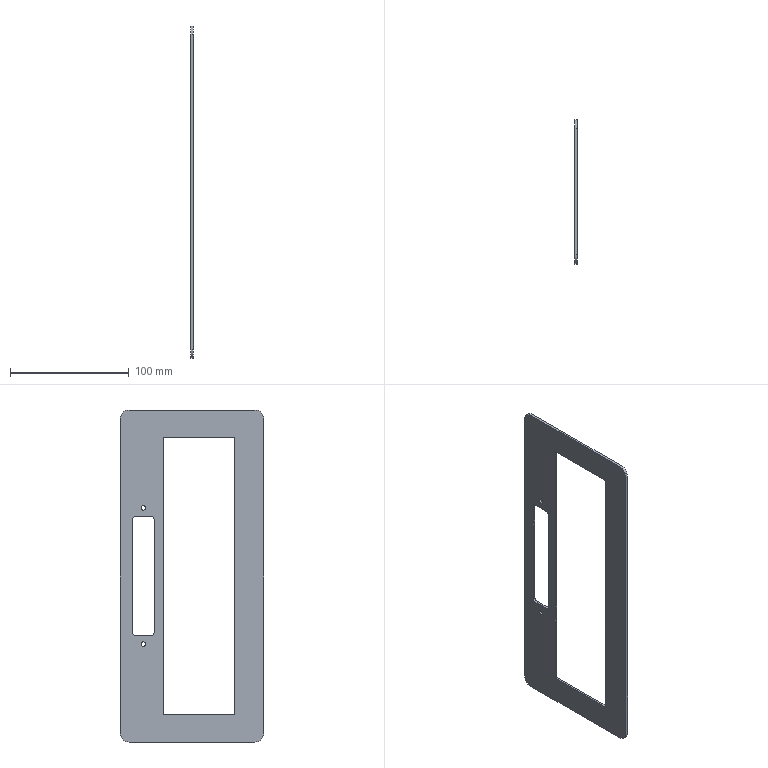Component | SolidWorks | YarnOutletAssembly-2_CashDispenserPanel-1 | 1 solid | 26 faces | box 2 x 121 x 280 mm | volume 35940 mm3 | plane 14 | cylinder 12 | commonest cylinder face diameters 4 x8 15 x4
STEP:
#1=CARTESIAN_POINT('',(-1.734,-15.239,2.343));
#2=VERTEX_POINT('',#1);
#3=CARTESIAN_POINT('',(-1.734,-15.239,2.185));
#4=VERTEX_POINT('',#3);
#5=CARTESIAN_POINT('',(-1.734,-15.239,2.264));
#6=DIRECTION('',(1.,0.,0.));
#7=DIRECTION('',(0.,0.,-1.));
#8=AXIS2_PLACEMENT_3D('',#5,#6,#7);
#9=CIRCLE('',#8,0.07874);
#10=EDGE_CURVE('',#2,#4,#9,.T.);
#11=ORIENTED_EDGE('',*,*,#10,.F.);
#12=CARTESIAN_POINT('',(-1.655,-15.239,2.343));
#13=VERTEX_POINT('',#12);
#14=CARTESIAN_POINT('',(-1.734,-15.239,2.343));
#15=DIRECTION('',(1.,0.,0.));
#16=VECTOR('',#15,39.37);
#17=LINE('',#14,#16);
#18=EDGE_CURVE('',#2,#13,#17,.T.);
#19=ORIENTED_EDGE('',*,*,#18,.T.);
#20=CARTESIAN_POINT('',(-1.655,-15.239,2.185));
#21=VERTEX_POINT('',#20);
#22=CARTESIAN_POINT('',(-1.655,-15.239,2.264));
#23=DIRECTION('',(1.,0.,0.));
#24=DIRECTION('',(0.,0.,-1.));
#25=AXIS2_PLACEMENT_3D('',#22,#23,#24);
#26=CIRCLE('',#25,0.07874);
#27=EDGE_CURVE('',#13,#21,#26,.T.);
#28=ORIENTED_EDGE('',*,*,#27,.T.);
#29=CARTESIAN_POINT('',(-1.734,-15.239,2.185));
#30=DIRECTION('',(1.,0.,0.));
#31=VECTOR('',#30,39.37);
#32=LINE('',#29,#31);
#33=EDGE_CURVE('',#4,#21,#32,.T.);
#34=ORIENTED_EDGE('',*,*,#33,.F.);
#35=EDGE_LOOP('',(#11,#19,#28,#34));
#36=FACE_OUTER_BOUND('',#35,.T.);
#37=CARTESIAN_POINT('',(-1.734,-15.239,2.264));
#38=DIRECTION('',(1.,0.,0.));
#39=DIRECTION('',(0.,0.,-1.));
#40=AXIS2_PLACEMENT_3D('',#37,#38,#39);
#41=CYLINDRICAL_SURFACE('',#40,0.07874);
#42=ADVANCED_FACE('',(#36),#41,.F.);
#43=CARTESIAN_POINT('',(-1.734,-15.239,-2.185));
#44=VERTEX_POINT('',#43);
#45=CARTESIAN_POINT('',(-1.734,-15.239,-2.343));
#46=VERTEX_POINT('',#45);
#47=CARTESIAN_POINT('',(-1.734,-15.239,-2.264));
#48=DIRECTION('',(1.,0.,0.));
#49=DIRECTION('',(0.,0.,-1.));
#50=AXIS2_PLACEMENT_3D('',#47,#48,#49);
#51=CIRCLE('',#50,0.07874);
#52=EDGE_CURVE('',#44,#46,#51,.T.);
#53=ORIENTED_EDGE('',*,*,#52,.F.);
#54=CARTESIAN_POINT('',(-1.655,-15.239,-2.185));
#55=VERTEX_POINT('',#54);
#56=CARTESIAN_POINT('',(-1.734,-15.239,-2.185));
#57=DIRECTION('',(1.,0.,0.));
#58=VECTOR('',#57,39.37);
#59=LINE('',#56,#58);
#60=EDGE_CURVE('',#44,#55,#59,.T.);
#61=ORIENTED_EDGE('',*,*,#60,.T.);
#62=CARTESIAN_POINT('',(-1.655,-15.239,-2.343));
#63=VERTEX_POINT('',#62);
#64=CARTESIAN_POINT('',(-1.655,-15.239,-2.264));
#65=DIRECTION('',(1.,0.,0.));
#66=DIRECTION('',(0.,0.,-1.));
#67=AXIS2_PLACEMENT_3D('',#64,#65,#66);
#68=CIRCLE('',#67,0.07874);
#69=EDGE_CURVE('',#55,#63,#68,.T.);
#70=ORIENTED_EDGE('',*,*,#69,.T.);
#71=CARTESIAN_POINT('',(-1.734,-15.239,-2.343));
#72=DIRECTION('',(1.,0.,0.));
#73=VECTOR('',#72,39.37);
#74=LINE('',#71,#73);
#75=EDGE_CURVE('',#46,#63,#74,.T.);
#76=ORIENTED_EDGE('',*,*,#75,.F.);
#77=EDGE_LOOP('',(#53,#61,#70,#76));
#78=FACE_OUTER_BOUND('',#77,.T.);
#79=CARTESIAN_POINT('',(-1.734,-15.239,-2.264));
#80=DIRECTION('',(1.,0.,0.));
#81=DIRECTION('',(0.,0.,-1.));
#82=AXIS2_PLACEMENT_3D('',#79,#80,#81);
#83=CYLINDRICAL_SURFACE('',#82,0.07874);
#84=ADVANCED_FACE('',(#78),#83,.F.);
#85=CARTESIAN_POINT('',(-1.655,-18.939,5.512));
#86=VERTEX_POINT('',#85);
#87=CARTESIAN_POINT('',(-1.655,-19.235,5.217));
#88=VERTEX_POINT('',#87);
#89=CARTESIAN_POINT('',(-1.655,-18.939,5.217));
#90=DIRECTION('',(1.,0.,0.));
#91=DIRECTION('',(0.,0.,-1.));
#92=AXIS2_PLACEMENT_3D('',#89,#90,#91);
#93=CIRCLE('',#92,0.2953);
#94=EDGE_CURVE('',#86,#88,#93,.T.);
#95=ORIENTED_EDGE('',*,*,#94,.F.);
#96=CARTESIAN_POINT('',(-1.734,-18.939,5.512));
#97=VERTEX_POINT('',#96);
#98=CARTESIAN_POINT('',(-1.734,-18.939,5.512));
#99=DIRECTION('',(1.,0.,0.));
#100=VECTOR('',#99,39.37);
#101=LINE('',#98,#100);
#102=EDGE_CURVE('',#97,#86,#101,.T.);
#103=ORIENTED_EDGE('',*,*,#102,.F.);
#104=CARTESIAN_POINT('',(-1.734,-19.235,5.217));
#105=VERTEX_POINT('',#104);
#106=CARTESIAN_POINT('',(-1.734,-18.939,5.217));
#107=DIRECTION('',(1.,0.,0.));
#108=DIRECTION('',(0.,0.,-1.));
#109=AXIS2_PLACEMENT_3D('',#106,#107,#108);
#110=CIRCLE('',#109,0.2953);
#111=EDGE_CURVE('',#97,#105,#110,.T.);
#112=ORIENTED_EDGE('',*,*,#111,.T.);
#113=CARTESIAN_POINT('',(-1.734,-19.235,5.217));
#114=DIRECTION('',(1.,0.,0.));
#115=VECTOR('',#114,39.37);
#116=LINE('',#113,#115);
#117=EDGE_CURVE('',#105,#88,#116,.T.);
#118=ORIENTED_EDGE('',*,*,#117,.T.);
#119=EDGE_LOOP('',(#95,#103,#112,#118));
#120=FACE_OUTER_BOUND('',#119,.T.);
#121=CARTESIAN_POINT('',(-1.734,-18.939,5.217));
#122=DIRECTION('',(1.,0.,0.));
#123=DIRECTION('',(0.,0.,-1.));
#124=AXIS2_PLACEMENT_3D('',#121,#122,#123);
#125=CYLINDRICAL_SURFACE('',#124,0.2953);
#126=ADVANCED_FACE('',(#120),#125,.T.);
#127=CARTESIAN_POINT('',(-1.655,-14.766,5.512));
#128=VERTEX_POINT('',#127);
#129=CARTESIAN_POINT('',(-1.655,-18.939,5.512));
#130=DIRECTION('',(0.,-1.,0.));
#131=VECTOR('',#130,39.37);
#132=LINE('',#129,#131);
#133=EDGE_CURVE('',#128,#86,#132,.T.);
#134=ORIENTED_EDGE('',*,*,#133,.F.);
#135=CARTESIAN_POINT('',(-1.734,-14.766,5.512));
#136=VERTEX_POINT('',#135);
#137=CARTESIAN_POINT('',(-1.734,-14.766,5.512));
#138=DIRECTION('',(1.,0.,0.));
#139=VECTOR('',#138,39.37);
#140=LINE('',#137,#139);
#141=EDGE_CURVE('',#136,#128,#140,.T.);
#142=ORIENTED_EDGE('',*,*,#141,.F.);
#143=CARTESIAN_POINT('',(-1.734,-18.939,5.512));
#144=DIRECTION('',(0.,-1.,0.));
#145=VECTOR('',#144,39.37);
#146=LINE('',#143,#145);
#147=EDGE_CURVE('',#136,#97,#146,.T.);
#148=ORIENTED_EDGE('',*,*,#147,.T.);
#149=ORIENTED_EDGE('',*,*,#102,.T.);
#150=EDGE_LOOP('',(#134,#142,#148,#149));
#151=FACE_OUTER_BOUND('',#150,.T.);
#152=CARTESIAN_POINT('',(-1.734,-18.939,5.512));
#153=DIRECTION('',(-0.,0.,1.));
#154=DIRECTION('',(1.,0.,0.));
#155=AXIS2_PLACEMENT_3D('',#152,#153,#154);
#156=PLANE('',#155);
#157=ADVANCED_FACE('',(#151),#156,.T.);
#158=CARTESIAN_POINT('',(-1.655,-14.471,5.217));
#159=VERTEX_POINT('',#158);
#160=CARTESIAN_POINT('',(-1.655,-14.766,5.217));
#161=DIRECTION('',(1.,0.,0.));
#162=DIRECTION('',(0.,0.,-1.));
#163=AXIS2_PLACEMENT_3D('',#160,#161,#162);
#164=CIRCLE('',#163,0.2953);
#165=EDGE_CURVE('',#159,#128,#164,.T.);
#166=ORIENTED_EDGE('',*,*,#165,.F.);
#167=CARTESIAN_POINT('',(-1.734,-14.471,5.217));
#168=VERTEX_POINT('',#167);
#169=CARTESIAN_POINT('',(-1.734,-14.471,5.217));
#170=DIRECTION('',(1.,0.,0.));
#171=VECTOR('',#170,39.37);
#172=LINE('',#169,#171);
#173=EDGE_CURVE('',#168,#159,#172,.T.);
#174=ORIENTED_EDGE('',*,*,#173,.F.);
#175=CARTESIAN_POINT('',(-1.734,-14.766,5.217));
#176=DIRECTION('',(1.,0.,0.));
#177=DIRECTION('',(0.,0.,-1.));
#178=AXIS2_PLACEMENT_3D('',#175,#176,#177);
#179=CIRCLE('',#178,0.2953);
#180=EDGE_CURVE('',#168,#136,#179,.T.);
#181=ORIENTED_EDGE('',*,*,#180,.T.);
#182=ORIENTED_EDGE('',*,*,#141,.T.);
#183=EDGE_LOOP('',(#166,#174,#181,#182));
#184=FACE_OUTER_BOUND('',#183,.T.);
#185=CARTESIAN_POINT('',(-1.734,-14.766,5.217));
#186=DIRECTION('',(1.,0.,0.));
#187=DIRECTION('',(0.,0.,-1.));
#188=AXIS2_PLACEMENT_3D('',#185,#186,#187);
#189=CYLINDRICAL_SURFACE('',#188,0.2953);
#190=ADVANCED_FACE('',(#184),#189,.T.);
#191=CARTESIAN_POINT('',(-1.655,-14.471,-5.217));
#192=VERTEX_POINT('',#191);
#193=CARTESIAN_POINT('',(-1.655,-14.471,5.217));
#194=DIRECTION('',(-0.,0.,1.));
#195=VECTOR('',#194,39.37);
#196=LINE('',#193,#195);
#197=EDGE_CURVE('',#192,#159,#196,.T.);
#198=ORIENTED_EDGE('',*,*,#197,.F.);
#199=CARTESIAN_POINT('',(-1.734,-14.471,-5.217));
#200=VERTEX_POINT('',#199);
#201=CARTESIAN_POINT('',(-1.734,-14.471,-5.217));
#202=DIRECTION('',(1.,0.,0.));
#203=VECTOR('',#202,39.37);
#204=LINE('',#201,#203);
#205=EDGE_CURVE('',#200,#192,#204,.T.);
#206=ORIENTED_EDGE('',*,*,#205,.F.);
#207=CARTESIAN_POINT('',(-1.734,-14.471,5.217));
#208=DIRECTION('',(-0.,0.,1.));
#209=VECTOR('',#208,39.37);
#210=LINE('',#207,#209);
#211=EDGE_CURVE('',#200,#168,#210,.T.);
#212=ORIENTED_EDGE('',*,*,#211,.T.);
#213=ORIENTED_EDGE('',*,*,#173,.T.);
#214=EDGE_LOOP('',(#198,#206,#212,#213));
#215=FACE_OUTER_BOUND('',#214,.T.);
#216=CARTESIAN_POINT('',(-1.734,-14.471,5.217));
#217=DIRECTION('',(-0.,1.,-0.));
#218=DIRECTION('',(1.,0.,0.));
#219=AXIS2_PLACEMENT_3D('',#216,#217,#218);
#220=PLANE('',#219);
#221=ADVANCED_FACE('',(#215),#220,.T.);
#222=CARTESIAN_POINT('',(-1.655,-14.766,-5.512));
#223=VERTEX_POINT('',#222);
#224=CARTESIAN_POINT('',(-1.655,-14.766,-5.217));
#225=DIRECTION('',(1.,0.,0.));
#226=DIRECTION('',(0.,0.,-1.));
#227=AXIS2_PLACEMENT_3D('',#224,#225,#226);
#228=CIRCLE('',#227,0.2953);
#229=EDGE_CURVE('',#223,#192,#228,.T.);
#230=ORIENTED_EDGE('',*,*,#229,.F.);
#231=CARTESIAN_POINT('',(-1.734,-14.766,-5.512));
#232=VERTEX_POINT('',#231);
#233=CARTESIAN_POINT('',(-1.734,-14.766,-5.512));
#234=DIRECTION('',(1.,0.,0.));
#235=VECTOR('',#234,39.37);
#236=LINE('',#233,#235);
#237=EDGE_CURVE('',#232,#223,#236,.T.);
#238=ORIENTED_EDGE('',*,*,#237,.F.);
#239=CARTESIAN_POINT('',(-1.734,-14.766,-5.217));
#240=DIRECTION('',(1.,0.,0.));
#241=DIRECTION('',(0.,0.,-1.));
#242=AXIS2_PLACEMENT_3D('',#239,#240,#241);
#243=CIRCLE('',#242,0.2953);
#244=EDGE_CURVE('',#232,#200,#243,.T.);
#245=ORIENTED_EDGE('',*,*,#244,.T.);
#246=ORIENTED_EDGE('',*,*,#205,.T.);
#247=EDGE_LOOP('',(#230,#238,#245,#246));
#248=FACE_OUTER_BOUND('',#247,.T.);
#249=CARTESIAN_POINT('',(-1.734,-14.766,-5.217));
#250=DIRECTION('',(1.,0.,0.));
#251=DIRECTION('',(0.,0.,-1.));
#252=AXIS2_PLACEMENT_3D('',#249,#250,#251);
#253=CYLINDRICAL_SURFACE('',#252,0.2953);
#254=ADVANCED_FACE('',(#248),#253,.T.);
#255=CARTESIAN_POINT('',(-1.655,-18.939,-5.512));
#256=VERTEX_POINT('',#255);
#257=CARTESIAN_POINT('',(-1.655,-18.939,-5.512));
#258=DIRECTION('',(-0.,1.,-0.));
#259=VECTOR('',#258,39.37);
#260=LINE('',#257,#259);
#261=EDGE_CURVE('',#256,#223,#260,.T.);
#262=ORIENTED_EDGE('',*,*,#261,.F.);
#263=CARTESIAN_POINT('',(-1.734,-18.939,-5.512));
#264=VERTEX_POINT('',#263);
#265=CARTESIAN_POINT('',(-1.734,-18.939,-5.512));
#266=DIRECTION('',(1.,0.,0.));
#267=VECTOR('',#266,39.37);
#268=LINE('',#265,#267);
#269=EDGE_CURVE('',#264,#256,#268,.T.);
#270=ORIENTED_EDGE('',*,*,#269,.F.);
#271=CARTESIAN_POINT('',(-1.734,-18.939,-5.512));
#272=DIRECTION('',(-0.,1.,-0.));
#273=VECTOR('',#272,39.37);
#274=LINE('',#271,#273);
#275=EDGE_CURVE('',#264,#232,#274,.T.);
#276=ORIENTED_EDGE('',*,*,#275,.T.);
#277=ORIENTED_EDGE('',*,*,#237,.T.);
#278=EDGE_LOOP('',(#262,#270,#276,#277));
#279=FACE_OUTER_BOUND('',#278,.T.);
#280=CARTESIAN_POINT('',(-1.734,-18.939,-5.512));
#281=DIRECTION('',(0.,-0.,-1.));
#282=DIRECTION('',(-1.,-0.,0.));
#283=AXIS2_PLACEMENT_3D('',#280,#281,#282);
#284=PLANE('',#283);
#285=ADVANCED_FACE('',(#279),#284,.T.);
#286=CARTESIAN_POINT('',(-1.655,-19.235,-5.217));
#287=VERTEX_POINT('',#286);
#288=CARTESIAN_POINT('',(-1.655,-18.939,-5.217));
#289=DIRECTION('',(1.,0.,0.));
#290=DIRECTION('',(0.,0.,-1.));
#291=AXIS2_PLACEMENT_3D('',#288,#289,#290);
#292=CIRCLE('',#291,0.2953);
#293=EDGE_CURVE('',#287,#256,#292,.T.);
#294=ORIENTED_EDGE('',*,*,#293,.F.);
#295=CARTESIAN_POINT('',(-1.734,-19.235,-5.217));
#296=VERTEX_POINT('',#295);
#297=CARTESIAN_POINT('',(-1.734,-19.235,-5.217));
#298=DIRECTION('',(1.,0.,0.));
#299=VECTOR('',#298,39.37);
#300=LINE('',#297,#299);
#301=EDGE_CURVE('',#296,#287,#300,.T.);
#302=ORIENTED_EDGE('',*,*,#301,.F.);
#303=CARTESIAN_POINT('',(-1.734,-18.939,-5.217));
#304=DIRECTION('',(1.,0.,0.));
#305=DIRECTION('',(0.,0.,-1.));
#306=AXIS2_PLACEMENT_3D('',#303,#304,#305);
#307=CIRCLE('',#306,0.2953);
#308=EDGE_CURVE('',#296,#264,#307,.T.);
#309=ORIENTED_EDGE('',*,*,#308,.T.);
#310=ORIENTED_EDGE('',*,*,#269,.T.);
#311=EDGE_LOOP('',(#294,#302,#309,#310));
#312=FACE_OUTER_BOUND('',#311,.T.);
#313=CARTESIAN_POINT('',(-1.734,-18.939,-5.217));
#314=DIRECTION('',(1.,0.,0.));
#315=DIRECTION('',(0.,0.,-1.));
#316=AXIS2_PLACEMENT_3D('',#313,#314,#315);
#317=CYLINDRICAL_SURFACE('',#316,0.2953);
#318=ADVANCED_FACE('',(#312),#317,.T.);
#319=CARTESIAN_POINT('',(-1.655,-19.235,5.217));
#320=DIRECTION('',(0.,-0.,-1.));
#321=VECTOR('',#320,39.37);
#322=LINE('',#319,#321);
#323=EDGE_CURVE('',#88,#287,#322,.T.);
#324=ORIENTED_EDGE('',*,*,#323,.F.);
#325=ORIENTED_EDGE('',*,*,#117,.F.);
#326=CARTESIAN_POINT('',(-1.734,-19.235,5.217));
#327=DIRECTION('',(0.,-0.,-1.));
#328=VECTOR('',#327,39.37);
#329=LINE('',#326,#328);
#330=EDGE_CURVE('',#105,#296,#329,.T.);
#331=ORIENTED_EDGE('',*,*,#330,.T.);
#332=ORIENTED_EDGE('',*,*,#301,.T.);
#333=EDGE_LOOP('',(#324,#325,#331,#332));
#334=FACE_OUTER_BOUND('',#333,.T.);
#335=CARTESIAN_POINT('',(-1.734,-19.235,5.217));
#336=DIRECTION('',(0.,-1.,0.));
#337=DIRECTION('',(-1.,-0.,0.));
#338=AXIS2_PLACEMENT_3D('',#335,#336,#337);
#339=PLANE('',#338);
#340=ADVANCED_FACE('',(#334),#339,.T.);
#341=CARTESIAN_POINT('',(-1.734,-15.239,2.264));
#342=DIRECTION('',(1.,0.,0.));
#343=DIRECTION('',(0.,0.,-1.));
#344=AXIS2_PLACEMENT_3D('',#341,#342,#343);
#345=CIRCLE('',#344,0.07874);
#346=EDGE_CURVE('',#4,#2,#345,.T.);
#347=ORIENTED_EDGE('',*,*,#346,.T.);
#348=ORIENTED_EDGE('',*,*,#10,.T.);
#349=EDGE_LOOP('',(#347,#348));
#350=FACE_BOUND('',#349,.T.);
#351=CARTESIAN_POINT('',(-1.734,-15.239,-2.264));
#352=DIRECTION('',(1.,0.,0.));
#353=DIRECTION('',(0.,0.,-1.));
#354=AXIS2_PLACEMENT_3D('',#351,#352,#353);
#355=CIRCLE('',#354,0.07874);
#356=EDGE_CURVE('',#46,#44,#355,.T.);
#357=ORIENTED_EDGE('',*,*,#356,.T.);
#358=ORIENTED_EDGE('',*,*,#52,.T.);
#359=EDGE_LOOP('',(#357,#358));
#360=FACE_BOUND('',#359,.T.);
#361=CARTESIAN_POINT('',(-1.734,-14.884,-1.89));
#362=VERTEX_POINT('',#361);
#363=CARTESIAN_POINT('',(-1.734,-14.884,1.89));
#364=VERTEX_POINT('',#363);
#365=CARTESIAN_POINT('',(-1.734,-14.884,-1.89));
#366=DIRECTION('',(-0.,0.,1.));
#367=VECTOR('',#366,39.37);
#368=LINE('',#365,#367);
#369=EDGE_CURVE('',#362,#364,#368,.T.);
#370=ORIENTED_EDGE('',*,*,#369,.T.);
#371=CARTESIAN_POINT('',(-1.734,-14.963,1.969));
#372=VERTEX_POINT('',#371);
#373=CARTESIAN_POINT('',(-1.734,-14.963,1.89));
#374=DIRECTION('',(1.,0.,0.));
#375=DIRECTION('',(0.,0.,-1.));
#376=AXIS2_PLACEMENT_3D('',#373,#374,#375);
#377=CIRCLE('',#376,0.07874);
#378=EDGE_CURVE('',#364,#372,#377,.T.);
#379=ORIENTED_EDGE('',*,*,#378,.T.);
#380=CARTESIAN_POINT('',(-1.734,-15.514,1.969));
#381=VERTEX_POINT('',#380);
#382=CARTESIAN_POINT('',(-1.734,-14.963,1.969));
#383=DIRECTION('',(0.,-1.,0.));
#384=VECTOR('',#383,39.37);
#385=LINE('',#382,#384);
#386=EDGE_CURVE('',#372,#381,#385,.T.);
#387=ORIENTED_EDGE('',*,*,#386,.T.);
#388=CARTESIAN_POINT('',(-1.734,-15.593,1.89));
#389=VERTEX_POINT('',#388);
#390=CARTESIAN_POINT('',(-1.734,-15.514,1.89));
#391=DIRECTION('',(1.,0.,0.));
#392=DIRECTION('',(0.,0.,-1.));
#393=AXIS2_PLACEMENT_3D('',#390,#391,#392);
#394=CIRCLE('',#393,0.07874);
#395=EDGE_CURVE('',#381,#389,#394,.T.);
#396=ORIENTED_EDGE('',*,*,#395,.T.);
#397=CARTESIAN_POINT('',(-1.734,-15.593,-1.89));
#398=VERTEX_POINT('',#397);
#399=CARTESIAN_POINT('',(-1.734,-15.593,1.89));
#400=DIRECTION('',(0.,-0.,-1.));
#401=VECTOR('',#400,39.37);
#402=LINE('',#399,#401);
#403=EDGE_CURVE('',#389,#398,#402,.T.);
#404=ORIENTED_EDGE('',*,*,#403,.T.);
#405=CARTESIAN_POINT('',(-1.734,-15.514,-1.969));
#406=VERTEX_POINT('',#405);
#407=CARTESIAN_POINT('',(-1.734,-15.514,-1.89));
#408=DIRECTION('',(1.,0.,0.));
#409=DIRECTION('',(0.,0.,-1.));
#410=AXIS2_PLACEMENT_3D('',#407,#408,#409);
#411=CIRCLE('',#410,0.07874);
#412=EDGE_CURVE('',#398,#406,#411,.T.);
#413=ORIENTED_EDGE('',*,*,#412,.T.);
#414=CARTESIAN_POINT('',(-1.734,-14.963,-1.969));
#415=VERTEX_POINT('',#414);
#416=CARTESIAN_POINT('',(-1.734,-15.514,-1.969));
#417=DIRECTION('',(-0.,1.,-0.));
#418=VECTOR('',#417,39.37);
#419=LINE('',#416,#418);
#420=EDGE_CURVE('',#406,#415,#419,.T.);
#421=ORIENTED_EDGE('',*,*,#420,.T.);
#422=CARTESIAN_POINT('',(-1.734,-14.963,-1.89));
#423=DIRECTION('',(1.,0.,0.));
#424=DIRECTION('',(0.,0.,-1.));
#425=AXIS2_PLACEMENT_3D('',#422,#423,#424);
#426=CIRCLE('',#425,0.07874);
#427=EDGE_CURVE('',#415,#362,#426,.T.);
#428=ORIENTED_EDGE('',*,*,#427,.T.);
#429=EDGE_LOOP('',(#370,#379,#387,#396,#404,#413,#421,#428));
#430=FACE_BOUND('',#429,.T.);
#431=CARTESIAN_POINT('',(-1.734,-18.27,-4.606));
#432=VERTEX_POINT('',#431);
#433=CARTESIAN_POINT('',(-1.734,-15.908,-4.606));
#434=VERTEX_POINT('',#433);
#435=CARTESIAN_POINT('',(-1.734,-18.27,-4.606));
#436=DIRECTION('',(-0.,1.,-0.));
#437=VECTOR('',#436,39.37);
#438=LINE('',#435,#437);
#439=EDGE_CURVE('',#432,#434,#438,.T.);
#440=ORIENTED_EDGE('',*,*,#439,.T.);
#441=CARTESIAN_POINT('',(-1.734,-15.908,4.606));
#442=VERTEX_POINT('',#441);
#443=CARTESIAN_POINT('',(-1.734,-15.908,-4.606));
#444=DIRECTION('',(-0.,0.,1.));
#445=VECTOR('',#444,39.37);
#446=LINE('',#443,#445);
#447=EDGE_CURVE('',#434,#442,#446,.T.);
#448=ORIENTED_EDGE('',*,*,#447,.T.);
#449=CARTESIAN_POINT('',(-1.734,-18.27,4.606));
#450=VERTEX_POINT('',#449);
#451=CARTESIAN_POINT('',(-1.734,-15.908,4.606));
#452=DIRECTION('',(0.,-1.,0.));
#453=VECTOR('',#452,39.37);
#454=LINE('',#451,#453);
#455=EDGE_CURVE('',#442,#450,#454,.T.);
#456=ORIENTED_EDGE('',*,*,#455,.T.);
#457=CARTESIAN_POINT('',(-1.734,-18.27,4.606));
#458=DIRECTION('',(0.,-0.,-1.));
#459=VECTOR('',#458,39.37);
#460=LINE('',#457,#459);
#461=EDGE_CURVE('',#450,#432,#460,.T.);
#462=ORIENTED_EDGE('',*,*,#461,.T.);
#463=EDGE_LOOP('',(#440,#448,#456,#462));
#464=FACE_BOUND('',#463,.T.);
#465=ORIENTED_EDGE('',*,*,#111,.F.);
#466=ORIENTED_EDGE('',*,*,#147,.F.);
#467=ORIENTED_EDGE('',*,*,#180,.F.);
#468=ORIENTED_EDGE('',*,*,#211,.F.);
#469=ORIENTED_EDGE('',*,*,#244,.F.);
#470=ORIENTED_EDGE('',*,*,#275,.F.);
#471=ORIENTED_EDGE('',*,*,#308,.F.);
#472=ORIENTED_EDGE('',*,*,#330,.F.);
#473=EDGE_LOOP('',(#465,#466,#467,#468,#469,#470,#471,#472));
#474=FACE_OUTER_BOUND('',#473,.T.);
#475=CARTESIAN_POINT('',(-1.734,-18.939,5.217));
#476=DIRECTION('',(1.,0.,0.));
#477=DIRECTION('',(0.,-0.,-1.));
#478=AXIS2_PLACEMENT_3D('',#475,#476,#477);
#479=PLANE('',#478);
#480=ADVANCED_FACE('',(#350,#360,#430,#464,#474),#479,.F.);
#481=CARTESIAN_POINT('',(-1.655,-15.239,2.264));
#482=DIRECTION('',(1.,0.,0.));
#483=DIRECTION('',(0.,0.,-1.));
#484=AXIS2_PLACEMENT_3D('',#481,#482,#483);
#485=CIRCLE('',#484,0.07874);
#486=EDGE_CURVE('',#21,#13,#485,.T.);
#487=ORIENTED_EDGE('',*,*,#486,.F.);
#488=ORIENTED_EDGE('',*,*,#27,.F.);
#489=EDGE_LOOP('',(#487,#488));
#490=FACE_BOUND('',#489,.T.);
#491=CARTESIAN_POINT('',(-1.655,-15.239,-2.264));
#492=DIRECTION('',(1.,0.,0.));
#493=DIRECTION('',(0.,0.,-1.));
#494=AXIS2_PLACEMENT_3D('',#491,#492,#493);
#495=CIRCLE('',#494,0.07874);
#496=EDGE_CURVE('',#63,#55,#495,.T.);
#497=ORIENTED_EDGE('',*,*,#496,.F.);
#498=ORIENTED_EDGE('',*,*,#69,.F.);
#499=EDGE_LOOP('',(#497,#498));
#500=FACE_BOUND('',#499,.T.);
#501=CARTESIAN_POINT('',(-1.655,-14.884,1.89));
#502=VERTEX_POINT('',#501);
#503=CARTESIAN_POINT('',(-1.655,-14.963,1.969));
#504=VERTEX_POINT('',#503);
#505=CARTESIAN_POINT('',(-1.655,-14.963,1.89));
#506=DIRECTION('',(1.,0.,0.));
#507=DIRECTION('',(0.,0.,-1.));
#508=AXIS2_PLACEMENT_3D('',#505,#506,#507);
#509=CIRCLE('',#508,0.07874);
#510=EDGE_CURVE('',#502,#504,#509,.T.);
#511=ORIENTED_EDGE('',*,*,#510,.F.);
#512=CARTESIAN_POINT('',(-1.655,-14.884,-1.89));
#513=VERTEX_POINT('',#512);
#514=CARTESIAN_POINT('',(-1.655,-14.884,-1.89));
#515=DIRECTION('',(-0.,0.,1.));
#516=VECTOR('',#515,39.37);
#517=LINE('',#514,#516);
#518=EDGE_CURVE('',#513,#502,#517,.T.);
#519=ORIENTED_EDGE('',*,*,#518,.F.);
#520=CARTESIAN_POINT('',(-1.655,-14.963,-1.969));
#521=VERTEX_POINT('',#520);
#522=CARTESIAN_POINT('',(-1.655,-14.963,-1.89));
#523=DIRECTION('',(1.,0.,0.));
#524=DIRECTION('',(0.,0.,-1.));
#525=AXIS2_PLACEMENT_3D('',#522,#523,#524);
#526=CIRCLE('',#525,0.07874);
#527=EDGE_CURVE('',#521,#513,#526,.T.);
#528=ORIENTED_EDGE('',*,*,#527,.F.);
#529=CARTESIAN_POINT('',(-1.655,-15.514,-1.969));
#530=VERTEX_POINT('',#529);
#531=CARTESIAN_POINT('',(-1.655,-15.514,-1.969));
#532=DIRECTION('',(-0.,1.,-0.));
#533=VECTOR('',#532,39.37);
#534=LINE('',#531,#533);
#535=EDGE_CURVE('',#530,#521,#534,.T.);
#536=ORIENTED_EDGE('',*,*,#535,.F.);
#537=CARTESIAN_POINT('',(-1.655,-15.593,-1.89));
#538=VERTEX_POINT('',#537);
#539=CARTESIAN_POINT('',(-1.655,-15.514,-1.89));
#540=DIRECTION('',(1.,0.,0.));
#541=DIRECTION('',(0.,0.,-1.));
#542=AXIS2_PLACEMENT_3D('',#539,#540,#541);
#543=CIRCLE('',#542,0.07874);
#544=EDGE_CURVE('',#538,#530,#543,.T.);
#545=ORIENTED_EDGE('',*,*,#544,.F.);
#546=CARTESIAN_POINT('',(-1.655,-15.593,1.89));
#547=VERTEX_POINT('',#546);
#548=CARTESIAN_POINT('',(-1.655,-15.593,1.89));
#549=DIRECTION('',(0.,-0.,-1.));
#550=VECTOR('',#549,39.37);
#551=LINE('',#548,#550);
#552=EDGE_CURVE('',#547,#538,#551,.T.);
#553=ORIENTED_EDGE('',*,*,#552,.F.);
#554=CARTESIAN_POINT('',(-1.655,-15.514,1.969));
#555=VERTEX_POINT('',#554);
#556=CARTESIAN_POINT('',(-1.655,-15.514,1.89));
#557=DIRECTION('',(1.,0.,0.));
#558=DIRECTION('',(0.,0.,-1.));
#559=AXIS2_PLACEMENT_3D('',#556,#557,#558);
#560=CIRCLE('',#559,0.07874);
#561=EDGE_CURVE('',#555,#547,#560,.T.);
#562=ORIENTED_EDGE('',*,*,#561,.F.);
#563=CARTESIAN_POINT('',(-1.655,-14.963,1.969));
#564=DIRECTION('',(0.,-1.,0.));
#565=VECTOR('',#564,39.37);
#566=LINE('',#563,#565);
#567=EDGE_CURVE('',#504,#555,#566,.T.);
#568=ORIENTED_EDGE('',*,*,#567,.F.);
#569=EDGE_LOOP('',(#511,#519,#528,#536,#545,#553,#562,#568));
#570=FACE_BOUND('',#569,.T.);
#571=CARTESIAN_POINT('',(-1.655,-15.908,-4.606));
#572=VERTEX_POINT('',#571);
#573=CARTESIAN_POINT('',(-1.655,-15.908,4.606));
#574=VERTEX_POINT('',#573);
#575=CARTESIAN_POINT('',(-1.655,-15.908,-4.606));
#576=DIRECTION('',(-0.,0.,1.));
#577=VECTOR('',#576,39.37);
#578=LINE('',#575,#577);
#579=EDGE_CURVE('',#572,#574,#578,.T.);
#580=ORIENTED_EDGE('',*,*,#579,.F.);
#581=CARTESIAN_POINT('',(-1.655,-18.27,-4.606));
#582=VERTEX_POINT('',#581);
#583=CARTESIAN_POINT('',(-1.655,-18.27,-4.606));
#584=DIRECTION('',(-0.,1.,-0.));
#585=VECTOR('',#584,39.37);
#586=LINE('',#583,#585);
#587=EDGE_CURVE('',#582,#572,#586,.T.);
#588=ORIENTED_EDGE('',*,*,#587,.F.);
#589=CARTESIAN_POINT('',(-1.655,-18.27,4.606));
#590=VERTEX_POINT('',#589);
#591=CARTESIAN_POINT('',(-1.655,-18.27,4.606));
#592=DIRECTION('',(0.,-0.,-1.));
#593=VECTOR('',#592,39.37);
#594=LINE('',#591,#593);
#595=EDGE_CURVE('',#590,#582,#594,.T.);
#596=ORIENTED_EDGE('',*,*,#595,.F.);
#597=CARTESIAN_POINT('',(-1.655,-15.908,4.606));
#598=DIRECTION('',(0.,-1.,0.));
#599=VECTOR('',#598,39.37);
#600=LINE('',#597,#599);
#601=EDGE_CURVE('',#574,#590,#600,.T.);
#602=ORIENTED_EDGE('',*,*,#601,.F.);
#603=EDGE_LOOP('',(#580,#588,#596,#602));
#604=FACE_BOUND('',#603,.T.);
#605=ORIENTED_EDGE('',*,*,#94,.T.);
#606=ORIENTED_EDGE('',*,*,#323,.T.);
#607=ORIENTED_EDGE('',*,*,#293,.T.);
#608=ORIENTED_EDGE('',*,*,#261,.T.);
#609=ORIENTED_EDGE('',*,*,#229,.T.);
#610=ORIENTED_EDGE('',*,*,#197,.T.);
#611=ORIENTED_EDGE('',*,*,#165,.T.);
#612=ORIENTED_EDGE('',*,*,#133,.T.);
#613=EDGE_LOOP('',(#605,#606,#607,#608,#609,#610,#611,#612));
#614=FACE_OUTER_BOUND('',#613,.T.);
#615=CARTESIAN_POINT('',(-1.655,-18.939,5.217));
#616=DIRECTION('',(1.,0.,0.));
#617=DIRECTION('',(0.,-0.,-1.));
#618=AXIS2_PLACEMENT_3D('',#615,#616,#617);
#619=PLANE('',#618);
#620=ADVANCED_FACE('',(#490,#500,#570,#604,#614),#619,.T.);
#621=ORIENTED_EDGE('',*,*,#579,.T.);
#622=CARTESIAN_POINT('',(-1.734,-15.908,4.606));
#623=DIRECTION('',(1.,0.,0.));
#624=VECTOR('',#623,39.37);
#625=LINE('',#622,#624);
#626=EDGE_CURVE('',#442,#574,#625,.T.);
#627=ORIENTED_EDGE('',*,*,#626,.F.);
#628=ORIENTED_EDGE('',*,*,#447,.F.);
#629=CARTESIAN_POINT('',(-1.734,-15.908,-4.606));
#630=DIRECTION('',(1.,0.,0.));
#631=VECTOR('',#630,39.37);
#632=LINE('',#629,#631);
#633=EDGE_CURVE('',#434,#572,#632,.T.);
#634=ORIENTED_EDGE('',*,*,#633,.T.);
#635=EDGE_LOOP('',(#621,#627,#628,#634));
#636=FACE_OUTER_BOUND('',#635,.T.);
#637=CARTESIAN_POINT('',(-1.734,-15.908,-4.606));
#638=DIRECTION('',(-0.,1.,-0.));
#639=DIRECTION('',(1.,0.,0.));
#640=AXIS2_PLACEMENT_3D('',#637,#638,#639);
#641=PLANE('',#640);
#642=ADVANCED_FACE('',(#636),#641,.F.);
#643=ORIENTED_EDGE('',*,*,#587,.T.);
#644=ORIENTED_EDGE('',*,*,#633,.F.);
#645=ORIENTED_EDGE('',*,*,#439,.F.);
#646=CARTESIAN_POINT('',(-1.734,-18.27,-4.606));
#647=DIRECTION('',(1.,0.,0.));
#648=VECTOR('',#647,39.37);
#649=LINE('',#646,#648);
#650=EDGE_CURVE('',#432,#582,#649,.T.);
#651=ORIENTED_EDGE('',*,*,#650,.T.);
#652=EDGE_LOOP('',(#643,#644,#645,#651));
#653=FACE_OUTER_BOUND('',#652,.T.);
#654=CARTESIAN_POINT('',(-1.734,-18.27,-4.606));
#655=DIRECTION('',(0.,-0.,-1.));
#656=DIRECTION('',(-1.,-0.,0.));
#657=AXIS2_PLACEMENT_3D('',#654,#655,#656);
#658=PLANE('',#657);
#659=ADVANCED_FACE('',(#653),#658,.F.);
#660=ORIENTED_EDGE('',*,*,#595,.T.);
#661=ORIENTED_EDGE('',*,*,#650,.F.);
#662=ORIENTED_EDGE('',*,*,#461,.F.);
#663=CARTESIAN_POINT('',(-1.734,-18.27,4.606));
#664=DIRECTION('',(1.,0.,0.));
#665=VECTOR('',#664,39.37);
#666=LINE('',#663,#665);
#667=EDGE_CURVE('',#450,#590,#666,.T.);
#668=ORIENTED_EDGE('',*,*,#667,.T.);
#669=EDGE_LOOP('',(#660,#661,#662,#668));
#670=FACE_OUTER_BOUND('',#669,.T.);
#671=CARTESIAN_POINT('',(-1.734,-18.27,4.606));
#672=DIRECTION('',(0.,-1.,0.));
#673=DIRECTION('',(-1.,-0.,0.));
#674=AXIS2_PLACEMENT_3D('',#671,#672,#673);
#675=PLANE('',#674);
#676=ADVANCED_FACE('',(#670),#675,.F.);
#677=ORIENTED_EDGE('',*,*,#601,.T.);
#678=ORIENTED_EDGE('',*,*,#667,.F.);
#679=ORIENTED_EDGE('',*,*,#455,.F.);
#680=ORIENTED_EDGE('',*,*,#626,.T.);
#681=EDGE_LOOP('',(#677,#678,#679,#680));
#682=FACE_OUTER_BOUND('',#681,.T.);
#683=CARTESIAN_POINT('',(-1.734,-15.908,4.606));
#684=DIRECTION('',(-0.,0.,1.));
#685=DIRECTION('',(1.,0.,0.));
#686=AXIS2_PLACEMENT_3D('',#683,#684,#685);
#687=PLANE('',#686);
#688=ADVANCED_FACE('',(#682),#687,.F.);
#689=ORIENTED_EDGE('',*,*,#510,.T.);
#690=CARTESIAN_POINT('',(-1.734,-14.963,1.969));
#691=DIRECTION('',(1.,0.,0.));
#692=VECTOR('',#691,39.37);
#693=LINE('',#690,#692);
#694=EDGE_CURVE('',#372,#504,#693,.T.);
#695=ORIENTED_EDGE('',*,*,#694,.F.);
#696=ORIENTED_EDGE('',*,*,#378,.F.);
#697=CARTESIAN_POINT('',(-1.734,-14.884,1.89));
#698=DIRECTION('',(1.,0.,0.));
#699=VECTOR('',#698,39.37);
#700=LINE('',#697,#699);
#701=EDGE_CURVE('',#364,#502,#700,.T.);
#702=ORIENTED_EDGE('',*,*,#701,.T.);
#703=EDGE_LOOP('',(#689,#695,#696,#702));
#704=FACE_OUTER_BOUND('',#703,.T.);
#705=CARTESIAN_POINT('',(-1.734,-14.963,1.89));
#706=DIRECTION('',(1.,0.,0.));
#707=DIRECTION('',(0.,0.,-1.));
#708=AXIS2_PLACEMENT_3D('',#705,#706,#707);
#709=CYLINDRICAL_SURFACE('',#708,0.07874);
#710=ADVANCED_FACE('',(#704),#709,.F.);
#711=ORIENTED_EDGE('',*,*,#518,.T.);
#712=ORIENTED_EDGE('',*,*,#701,.F.);
#713=ORIENTED_EDGE('',*,*,#369,.F.);
#714=CARTESIAN_POINT('',(-1.734,-14.884,-1.89));
#715=DIRECTION('',(1.,0.,0.));
#716=VECTOR('',#715,39.37);
#717=LINE('',#714,#716);
#718=EDGE_CURVE('',#362,#513,#717,.T.);
#719=ORIENTED_EDGE('',*,*,#718,.T.);
#720=EDGE_LOOP('',(#711,#712,#713,#719));
#721=FACE_OUTER_BOUND('',#720,.T.);
#722=CARTESIAN_POINT('',(-1.734,-14.884,-1.89));
#723=DIRECTION('',(-0.,1.,-0.));
#724=DIRECTION('',(1.,0.,0.));
#725=AXIS2_PLACEMENT_3D('',#722,#723,#724);
#726=PLANE('',#725);
#727=ADVANCED_FACE('',(#721),#726,.F.);
#728=ORIENTED_EDGE('',*,*,#527,.T.);
#729=ORIENTED_EDGE('',*,*,#718,.F.);
#730=ORIENTED_EDGE('',*,*,#427,.F.);
#731=CARTESIAN_POINT('',(-1.734,-14.963,-1.969));
#732=DIRECTION('',(1.,0.,0.));
#733=VECTOR('',#732,39.37);
#734=LINE('',#731,#733);
#735=EDGE_CURVE('',#415,#521,#734,.T.);
#736=ORIENTED_EDGE('',*,*,#735,.T.);
#737=EDGE_LOOP('',(#728,#729,#730,#736));
#738=FACE_OUTER_BOUND('',#737,.T.);
#739=CARTESIAN_POINT('',(-1.734,-14.963,-1.89));
#740=DIRECTION('',(1.,0.,0.));
#741=DIRECTION('',(0.,0.,-1.));
#742=AXIS2_PLACEMENT_3D('',#739,#740,#741);
#743=CYLINDRICAL_SURFACE('',#742,0.07874);
#744=ADVANCED_FACE('',(#738),#743,.F.);
#745=ORIENTED_EDGE('',*,*,#535,.T.);
#746=ORIENTED_EDGE('',*,*,#735,.F.);
#747=ORIENTED_EDGE('',*,*,#420,.F.);
#748=CARTESIAN_POINT('',(-1.734,-15.514,-1.969));
#749=DIRECTION('',(1.,0.,0.));
#750=VECTOR('',#749,39.37);
#751=LINE('',#748,#750);
#752=EDGE_CURVE('',#406,#530,#751,.T.);
#753=ORIENTED_EDGE('',*,*,#752,.T.);
#754=EDGE_LOOP('',(#745,#746,#747,#753));
#755=FACE_OUTER_BOUND('',#754,.T.);
#756=CARTESIAN_POINT('',(-1.734,-15.514,-1.969));
#757=DIRECTION('',(0.,-0.,-1.));
#758=DIRECTION('',(-1.,-0.,0.));
#759=AXIS2_PLACEMENT_3D('',#756,#757,#758);
#760=PLANE('',#759);
#761=ADVANCED_FACE('',(#755),#760,.F.);
#762=ORIENTED_EDGE('',*,*,#544,.T.);
#763=ORIENTED_EDGE('',*,*,#752,.F.);
#764=ORIENTED_EDGE('',*,*,#412,.F.);
#765=CARTESIAN_POINT('',(-1.734,-15.593,-1.89));
#766=DIRECTION('',(1.,0.,0.));
#767=VECTOR('',#766,39.37);
#768=LINE('',#765,#767);
#769=EDGE_CURVE('',#398,#538,#768,.T.);
#770=ORIENTED_EDGE('',*,*,#769,.T.);
#771=EDGE_LOOP('',(#762,#763,#764,#770));
#772=FACE_OUTER_BOUND('',#771,.T.);
#773=CARTESIAN_POINT('',(-1.734,-15.514,-1.89));
#774=DIRECTION('',(1.,0.,0.));
#775=DIRECTION('',(0.,0.,-1.));
#776=AXIS2_PLACEMENT_3D('',#773,#774,#775);
#777=CYLINDRICAL_SURFACE('',#776,0.07874);
#778=ADVANCED_FACE('',(#772),#777,.F.);
#779=ORIENTED_EDGE('',*,*,#552,.T.);
#780=ORIENTED_EDGE('',*,*,#769,.F.);
#781=ORIENTED_EDGE('',*,*,#403,.F.);
#782=CARTESIAN_POINT('',(-1.734,-15.593,1.89));
#783=DIRECTION('',(1.,0.,0.));
#784=VECTOR('',#783,39.37);
#785=LINE('',#782,#784);
#786=EDGE_CURVE('',#389,#547,#785,.T.);
#787=ORIENTED_EDGE('',*,*,#786,.T.);
#788=EDGE_LOOP('',(#779,#780,#781,#787));
#789=FACE_OUTER_BOUND('',#788,.T.);
#790=CARTESIAN_POINT('',(-1.734,-15.593,1.89));
#791=DIRECTION('',(0.,-1.,0.));
#792=DIRECTION('',(-1.,-0.,0.));
#793=AXIS2_PLACEMENT_3D('',#790,#791,#792);
#794=PLANE('',#793);
#795=ADVANCED_FACE('',(#789),#794,.F.);
#796=ORIENTED_EDGE('',*,*,#561,.T.);
#797=ORIENTED_EDGE('',*,*,#786,.F.);
#798=ORIENTED_EDGE('',*,*,#395,.F.);
#799=CARTESIAN_POINT('',(-1.734,-15.514,1.969));
#800=DIRECTION('',(1.,0.,0.));
#801=VECTOR('',#800,39.37);
#802=LINE('',#799,#801);
#803=EDGE_CURVE('',#381,#555,#802,.T.);
#804=ORIENTED_EDGE('',*,*,#803,.T.);
#805=EDGE_LOOP('',(#796,#797,#798,#804));
#806=FACE_OUTER_BOUND('',#805,.T.);
#807=CARTESIAN_POINT('',(-1.734,-15.514,1.89));
#808=DIRECTION('',(1.,0.,0.));
#809=DIRECTION('',(0.,0.,-1.));
#810=AXIS2_PLACEMENT_3D('',#807,#808,#809);
#811=CYLINDRICAL_SURFACE('',#810,0.07874);
#812=ADVANCED_FACE('',(#806),#811,.F.);
#813=ORIENTED_EDGE('',*,*,#567,.T.);
#814=ORIENTED_EDGE('',*,*,#803,.F.);
#815=ORIENTED_EDGE('',*,*,#386,.F.);
#816=ORIENTED_EDGE('',*,*,#694,.T.);
#817=EDGE_LOOP('',(#813,#814,#815,#816));
#818=FACE_OUTER_BOUND('',#817,.T.);
#819=CARTESIAN_POINT('',(-1.734,-14.963,1.969));
#820=DIRECTION('',(-0.,0.,1.));
#821=DIRECTION('',(1.,0.,0.));
#822=AXIS2_PLACEMENT_3D('',#819,#820,#821);
#823=PLANE('',#822);
#824=ADVANCED_FACE('',(#818),#823,.F.);
#825=ORIENTED_EDGE('',*,*,#60,.F.);
#826=ORIENTED_EDGE('',*,*,#356,.F.);
#827=ORIENTED_EDGE('',*,*,#75,.T.);
#828=ORIENTED_EDGE('',*,*,#496,.T.);
#829=EDGE_LOOP('',(#825,#826,#827,#828));
#830=FACE_OUTER_BOUND('',#829,.T.);
#831=CARTESIAN_POINT('',(-1.734,-15.239,-2.264));
#832=DIRECTION('',(1.,0.,0.));
#833=DIRECTION('',(0.,0.,-1.));
#834=AXIS2_PLACEMENT_3D('',#831,#832,#833);
#835=CYLINDRICAL_SURFACE('',#834,0.07874);
#836=ADVANCED_FACE('',(#830),#835,.F.);
#837=ORIENTED_EDGE('',*,*,#18,.F.);
#838=ORIENTED_EDGE('',*,*,#346,.F.);
#839=ORIENTED_EDGE('',*,*,#33,.T.);
#840=ORIENTED_EDGE('',*,*,#486,.T.);
#841=EDGE_LOOP('',(#837,#838,#839,#840));
#842=FACE_OUTER_BOUND('',#841,.T.);
#843=CARTESIAN_POINT('',(-1.734,-15.239,2.264));
#844=DIRECTION('',(1.,0.,0.));
#845=DIRECTION('',(0.,0.,-1.));
#846=AXIS2_PLACEMENT_3D('',#843,#844,#845);
#847=CYLINDRICAL_SURFACE('',#846,0.07874);
#848=ADVANCED_FACE('',(#842),#847,.F.);
#849=CLOSED_SHELL('',(#42,#84,#126,#157,#190,#221,#254,#285,#318,#340,#480,#620,#642,#659,#676,#688,#710,#727,#744,#761,#778,#795,#812,#824,#836,#848));
#850=MANIFOLD_SOLID_BREP('',#849);
#851=CARTESIAN_POINT('',(0.,0.,0.));
#852=DIRECTION('',(0.,0.,1.));
#853=DIRECTION('',(1.,0.,0.));
#854=AXIS2_PLACEMENT_3D('',#851,#852,#853);
#855=(LENGTH_UNIT()NAMED_UNIT(*)SI_UNIT($,.METRE.));
#856=LENGTH_MEASURE_WITH_UNIT(LENGTH_MEASURE(0.0254),#855);
#857=DIMENSIONAL_EXPONENTS(1.,0.,0.,0.,0.,0.,0.);
#858=(CONVERSION_BASED_UNIT('',#856)LENGTH_UNIT()NAMED_UNIT(#857));
#859=UNCERTAINTY_MEASURE_WITH_UNIT(LENGTH_MEASURE(0.00001),#858,'','');
#860=(NAMED_UNIT(*)PLANE_ANGLE_UNIT()SI_UNIT($,.RADIAN.));
#861=(NAMED_UNIT(*)SI_UNIT($,.STERADIAN.)SOLID_ANGLE_UNIT());
#862=(GEOMETRIC_REPRESENTATION_CONTEXT(3)GLOBAL_UNCERTAINTY_ASSIGNED_CONTEXT((#859))GLOBAL_UNIT_ASSIGNED_CONTEXT((#858,#860,#861))REPRESENTATION_CONTEXT('',''));
#863=ADVANCED_BREP_SHAPE_REPRESENTATION('',(#850,#854),#862);
#864=COLOUR_RGB('',0.7922,0.8196,0.9333);
#865=FILL_AREA_STYLE_COLOUR('',#864);
#866=FILL_AREA_STYLE('',(#865));
#867=SURFACE_STYLE_FILL_AREA(#866);
#868=SURFACE_SIDE_STYLE('',(#867));
#869=SURFACE_STYLE_USAGE(.BOTH.,#868);
#870=PRESENTATION_STYLE_ASSIGNMENT((#869));
#871=STYLED_ITEM('',(#870),#850);
#872=PRESENTATION_LAYER_ASSIGNMENT('','',(#871));
#873=(LENGTH_UNIT()NAMED_UNIT(*)SI_UNIT($,.METRE.));
#874=LENGTH_MEASURE_WITH_UNIT(LENGTH_MEASURE(0.0254),#873);
#875=DIMENSIONAL_EXPONENTS(1.,0.,0.,0.,0.,0.,0.);
#876=(CONVERSION_BASED_UNIT('',#874)LENGTH_UNIT()NAMED_UNIT(#875));
#877=UNCERTAINTY_MEASURE_WITH_UNIT(LENGTH_MEASURE(0.00001),#876,'','');
#878=(NAMED_UNIT(*)PLANE_ANGLE_UNIT()SI_UNIT($,.RADIAN.));
#879=(NAMED_UNIT(*)SI_UNIT($,.STERADIAN.)SOLID_ANGLE_UNIT());
#880=(GEOMETRIC_REPRESENTATION_CONTEXT(3)GLOBAL_UNCERTAINTY_ASSIGNED_CONTEXT((#877))GLOBAL_UNIT_ASSIGNED_CONTEXT((#876,#878,#879))REPRESENTATION_CONTEXT('',''));
#881=MECHANICAL_DESIGN_GEOMETRIC_PRESENTATION_REPRESENTATION('',(#871),#880);